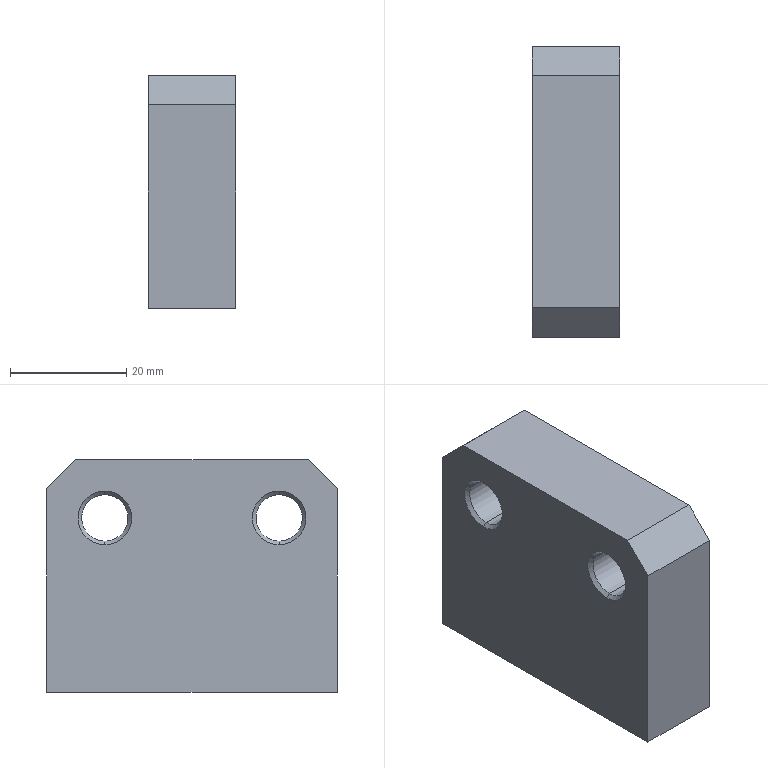Component | SolidWorks | DoubleFilmTransport-1_PositioningScrewPlate-1 | 1 solid | 28 faces | box 15 x 50 x 40 mm | volume 27415 mm3 | cone 12 | cylinder 8 | plane 8 | commonest cylinder face diameters 5 x4 8 x4
build123d program:
from build123d import *

# Parameters (mm, degrees)
SKETCH1_W                    = 40
SKETCH1_H                    = 50
BOSS_EXTRUDE1_DEPTH          = 15
F_6_8_6_8_DIAMETER_HOLE1_D   = 8
F_5_0_5_DIAMETER_HOLE1_D     = 5
F_5_0_5_DIAMETER_HOLE1_DEPTH = 17
F_5_0_5_DIAMETER_HOLE1_TIP   = 1.502
CHAMFER1_SIZE                = 0.625
CHAMFER2_SIZE                = 0.525
CHAMFER3_SIZE                = 5


with BuildPart() as part:
    # Sketch1 → Boss-Extrude1 (new body)
    with BuildSketch(Plane.XY.offset(7.5)):
        with Locations((20, 0)):
            Rectangle(SKETCH1_W, SKETCH1_H)
    extrude(amount=-BOSS_EXTRUDE1_DEPTH)

    # 6.8 _6.8_ Diameter Hole1 (through all)
    with Locations(Plane.XY.offset(7.5)):
        with Locations((30, -15), (30, 15)):
            Hole(F_6_8_6_8_DIAMETER_HOLE1_D / 2)

    # 5.0 _5_ Diameter Hole1
    with Locations(Plane.ZY):
        with Locations((0, -15), (0, 15)):
            Hole(F_5_0_5_DIAMETER_HOLE1_D / 2, depth=F_5_0_5_DIAMETER_HOLE1_DEPTH)
            with Locations((0, 0, -(F_5_0_5_DIAMETER_HOLE1_DEPTH + F_5_0_5_DIAMETER_HOLE1_TIP / 2))):  # 118° drill point
                Cone(0, F_5_0_5_DIAMETER_HOLE1_D / 2, F_5_0_5_DIAMETER_HOLE1_TIP, mode=Mode.SUBTRACT)

    # Chamfer1
    chamfer1_edges = [part.edges().sort_by_distance(p)[0] for p in [
        (34, 15, 7.5),
        (34, -15, 7.5),
    ]]
    chamfer(chamfer1_edges, length=CHAMFER1_SIZE)

    # Chamfer2
    chamfer2_edges = [part.edges().sort_by_distance(p)[0] for p in [
        (0, 15, 2.5),
        (0, -15, 2.5),
    ]]
    chamfer(chamfer2_edges, length=CHAMFER2_SIZE)

    # Chamfer3
    chamfer3_edges = [part.edges().sort_by_distance(p)[0] for p in [
        (40, 25, 0),
        (40, -25, 0),
    ]]
    chamfer(chamfer3_edges, length=CHAMFER3_SIZE)


solid = part.part

# Placed as in the assembly
solid = solid.moved(Location((-298.746, 150.373, -16.5), (0, -90, 0)))
STEP:
#1=CARTESIAN_POINT('',(-11.663,5.33,-0.6289));
#2=VERTEX_POINT('',#1);
#3=CARTESIAN_POINT('',(-11.86,5.33,-0.6289));
#4=VERTEX_POINT('',#3);
#5=CARTESIAN_POINT('',(-11.762,5.33,-0.6289));
#6=DIRECTION('',(0.,0.,-1.));
#7=DIRECTION('',(-1.,0.,0.));
#8=AXIS2_PLACEMENT_3D('',#5,#6,#7);
#9=CIRCLE('',#8,0.09843);
#10=EDGE_CURVE('',#2,#4,#9,.T.);
#11=ORIENTED_EDGE('',*,*,#10,.F.);
#12=CARTESIAN_POINT('',(-11.643,5.33,-0.6496));
#13=VERTEX_POINT('',#12);
#14=CARTESIAN_POINT('',(-11.663,5.33,-0.6289));
#15=DIRECTION('',(0.7071,0.,-0.7071));
#16=VECTOR('',#15,39.37);
#17=LINE('',#14,#16);
#18=EDGE_CURVE('',#2,#13,#17,.T.);
#19=ORIENTED_EDGE('',*,*,#18,.T.);
#20=CARTESIAN_POINT('',(-11.881,5.33,-0.6496));
#21=VERTEX_POINT('',#20);
#22=CARTESIAN_POINT('',(-11.762,5.33,-0.6496));
#23=DIRECTION('',(0.,-0.,1.));
#24=DIRECTION('',(0.,-1.,0.));
#25=AXIS2_PLACEMENT_3D('',#22,#23,#24);
#26=CIRCLE('',#25,0.1191);
#27=EDGE_CURVE('',#21,#13,#26,.T.);
#28=ORIENTED_EDGE('',*,*,#27,.F.);
#29=CARTESIAN_POINT('',(-11.86,5.33,-0.6289));
#30=DIRECTION('',(-0.7071,0.,-0.7071));
#31=VECTOR('',#30,39.37);
#32=LINE('',#29,#31);
#33=EDGE_CURVE('',#4,#21,#32,.T.);
#34=ORIENTED_EDGE('',*,*,#33,.F.);
#35=EDGE_LOOP('',(#11,#19,#28,#34));
#36=FACE_OUTER_BOUND('',#35,.T.);
#37=CARTESIAN_POINT('',(-11.762,5.33,-0.6289));
#38=DIRECTION('',(0.,0.,-1.));
#39=DIRECTION('',(-1.,0.,0.));
#40=AXIS2_PLACEMENT_3D('',#37,#38,#39);
#41=CONICAL_SURFACE('',#40,0.09843,0.7854);
#42=ADVANCED_FACE('',(#36),#41,.F.);
#43=CARTESIAN_POINT('',(-11.663,6.511,-0.6289));
#44=VERTEX_POINT('',#43);
#45=CARTESIAN_POINT('',(-11.86,6.511,-0.6289));
#46=VERTEX_POINT('',#45);
#47=CARTESIAN_POINT('',(-11.762,6.511,-0.6289));
#48=DIRECTION('',(0.,0.,-1.));
#49=DIRECTION('',(-1.,0.,0.));
#50=AXIS2_PLACEMENT_3D('',#47,#48,#49);
#51=CIRCLE('',#50,0.09843);
#52=EDGE_CURVE('',#44,#46,#51,.T.);
#53=ORIENTED_EDGE('',*,*,#52,.F.);
#54=CARTESIAN_POINT('',(-11.643,6.511,-0.6496));
#55=VERTEX_POINT('',#54);
#56=CARTESIAN_POINT('',(-11.663,6.511,-0.6289));
#57=DIRECTION('',(0.7071,0.,-0.7071));
#58=VECTOR('',#57,39.37);
#59=LINE('',#56,#58);
#60=EDGE_CURVE('',#44,#55,#59,.T.);
#61=ORIENTED_EDGE('',*,*,#60,.T.);
#62=CARTESIAN_POINT('',(-11.881,6.511,-0.6496));
#63=VERTEX_POINT('',#62);
#64=CARTESIAN_POINT('',(-11.762,6.511,-0.6496));
#65=DIRECTION('',(0.,-0.,1.));
#66=DIRECTION('',(0.,-1.,0.));
#67=AXIS2_PLACEMENT_3D('',#64,#65,#66);
#68=CIRCLE('',#67,0.1191);
#69=EDGE_CURVE('',#63,#55,#68,.T.);
#70=ORIENTED_EDGE('',*,*,#69,.F.);
#71=CARTESIAN_POINT('',(-11.86,6.511,-0.6289));
#72=DIRECTION('',(-0.7071,0.,-0.7071));
#73=VECTOR('',#72,39.37);
#74=LINE('',#71,#73);
#75=EDGE_CURVE('',#46,#63,#74,.T.);
#76=ORIENTED_EDGE('',*,*,#75,.F.);
#77=EDGE_LOOP('',(#53,#61,#70,#76));
#78=FACE_OUTER_BOUND('',#77,.T.);
#79=CARTESIAN_POINT('',(-11.762,6.511,-0.6289));
#80=DIRECTION('',(0.,0.,-1.));
#81=DIRECTION('',(-1.,0.,0.));
#82=AXIS2_PLACEMENT_3D('',#79,#80,#81);
#83=CONICAL_SURFACE('',#82,0.09843,0.7854);
#84=ADVANCED_FACE('',(#78),#83,.F.);
#85=CARTESIAN_POINT('',(-12.032,5.33,0.374));
#86=VERTEX_POINT('',#85);
#87=CARTESIAN_POINT('',(-12.032,5.33,0.689));
#88=VERTEX_POINT('',#87);
#89=CARTESIAN_POINT('',(-12.032,5.33,0.5315));
#90=DIRECTION('',(-1.,0.,0.));
#91=DIRECTION('',(0.,0.,1.));
#92=AXIS2_PLACEMENT_3D('',#89,#90,#91);
#93=CIRCLE('',#92,0.1575);
#94=EDGE_CURVE('',#86,#88,#93,.T.);
#95=ORIENTED_EDGE('',*,*,#94,.F.);
#96=CARTESIAN_POINT('',(-12.057,5.33,0.3494));
#97=VERTEX_POINT('',#96);
#98=CARTESIAN_POINT('',(-12.032,5.33,0.374));
#99=DIRECTION('',(-0.7071,0.,-0.7071));
#100=VECTOR('',#99,39.37);
#101=LINE('',#98,#100);
#102=EDGE_CURVE('',#86,#97,#101,.T.);
#103=ORIENTED_EDGE('',*,*,#102,.T.);
#104=CARTESIAN_POINT('',(-12.057,5.33,0.7136));
#105=VERTEX_POINT('',#104);
#106=CARTESIAN_POINT('',(-12.057,5.33,0.5315));
#107=DIRECTION('',(1.,0.,0.));
#108=DIRECTION('',(0.,0.,1.));
#109=AXIS2_PLACEMENT_3D('',#106,#107,#108);
#110=CIRCLE('',#109,0.1821);
#111=EDGE_CURVE('',#105,#97,#110,.T.);
#112=ORIENTED_EDGE('',*,*,#111,.F.);
#113=CARTESIAN_POINT('',(-12.032,5.33,0.689));
#114=DIRECTION('',(-0.7071,0.,0.7071));
#115=VECTOR('',#114,39.37);
#116=LINE('',#113,#115);
#117=EDGE_CURVE('',#88,#105,#116,.T.);
#118=ORIENTED_EDGE('',*,*,#117,.F.);
#119=EDGE_LOOP('',(#95,#103,#112,#118));
#120=FACE_OUTER_BOUND('',#119,.T.);
#121=CARTESIAN_POINT('',(-12.032,5.33,0.5315));
#122=DIRECTION('',(-1.,0.,0.));
#123=DIRECTION('',(0.,0.,1.));
#124=AXIS2_PLACEMENT_3D('',#121,#122,#123);
#125=CONICAL_SURFACE('',#124,0.1575,0.7854);
#126=ADVANCED_FACE('',(#120),#125,.F.);
#127=CARTESIAN_POINT('',(-12.032,6.511,0.374));
#128=VERTEX_POINT('',#127);
#129=CARTESIAN_POINT('',(-12.032,6.511,0.689));
#130=VERTEX_POINT('',#129);
#131=CARTESIAN_POINT('',(-12.032,6.511,0.5315));
#132=DIRECTION('',(-1.,0.,0.));
#133=DIRECTION('',(0.,0.,1.));
#134=AXIS2_PLACEMENT_3D('',#131,#132,#133);
#135=CIRCLE('',#134,0.1575);
#136=EDGE_CURVE('',#128,#130,#135,.T.);
#137=ORIENTED_EDGE('',*,*,#136,.F.);
#138=CARTESIAN_POINT('',(-12.057,6.511,0.3494));
#139=VERTEX_POINT('',#138);
#140=CARTESIAN_POINT('',(-12.032,6.511,0.374));
#141=DIRECTION('',(-0.7071,0.,-0.7071));
#142=VECTOR('',#141,39.37);
#143=LINE('',#140,#142);
#144=EDGE_CURVE('',#128,#139,#143,.T.);
#145=ORIENTED_EDGE('',*,*,#144,.T.);
#146=CARTESIAN_POINT('',(-12.057,6.511,0.7136));
#147=VERTEX_POINT('',#146);
#148=CARTESIAN_POINT('',(-12.057,6.511,0.5315));
#149=DIRECTION('',(1.,0.,0.));
#150=DIRECTION('',(0.,0.,1.));
#151=AXIS2_PLACEMENT_3D('',#148,#149,#150);
#152=CIRCLE('',#151,0.1821);
#153=EDGE_CURVE('',#147,#139,#152,.T.);
#154=ORIENTED_EDGE('',*,*,#153,.F.);
#155=CARTESIAN_POINT('',(-12.032,6.511,0.689));
#156=DIRECTION('',(-0.7071,0.,0.7071));
#157=VECTOR('',#156,39.37);
#158=LINE('',#155,#157);
#159=EDGE_CURVE('',#130,#147,#158,.T.);
#160=ORIENTED_EDGE('',*,*,#159,.F.);
#161=EDGE_LOOP('',(#137,#145,#154,#160));
#162=FACE_OUTER_BOUND('',#161,.T.);
#163=CARTESIAN_POINT('',(-12.032,6.511,0.5315));
#164=DIRECTION('',(-1.,0.,0.));
#165=DIRECTION('',(0.,0.,1.));
#166=AXIS2_PLACEMENT_3D('',#163,#164,#165);
#167=CONICAL_SURFACE('',#166,0.1575,0.7854);
#168=ADVANCED_FACE('',(#162),#167,.F.);
#169=CARTESIAN_POINT('',(-11.663,5.33,0.01969));
#170=VERTEX_POINT('',#169);
#171=CARTESIAN_POINT('',(-11.86,5.33,0.01969));
#172=VERTEX_POINT('',#171);
#173=CARTESIAN_POINT('',(-11.762,5.33,0.01969));
#174=DIRECTION('',(0.,0.,-1.));
#175=DIRECTION('',(-1.,0.,0.));
#176=AXIS2_PLACEMENT_3D('',#173,#174,#175);
#177=CIRCLE('',#176,0.09843);
#178=EDGE_CURVE('',#170,#172,#177,.T.);
#179=ORIENTED_EDGE('',*,*,#178,.F.);
#180=CARTESIAN_POINT('',(-11.663,5.33,-0.6496));
#181=DIRECTION('',(0.,0.,-1.));
#182=VECTOR('',#181,39.37);
#183=LINE('',#180,#182);
#184=EDGE_CURVE('',#170,#2,#183,.T.);
#185=ORIENTED_EDGE('',*,*,#184,.T.);
#186=ORIENTED_EDGE('',*,*,#10,.T.);
#187=CARTESIAN_POINT('',(-11.86,5.33,-0.6496));
#188=DIRECTION('',(0.,0.,-1.));
#189=VECTOR('',#188,39.37);
#190=LINE('',#187,#189);
#191=EDGE_CURVE('',#172,#4,#190,.T.);
#192=ORIENTED_EDGE('',*,*,#191,.F.);
#193=EDGE_LOOP('',(#179,#185,#186,#192));
#194=FACE_OUTER_BOUND('',#193,.T.);
#195=CARTESIAN_POINT('',(-11.762,5.33,-0.6496));
#196=DIRECTION('',(0.,0.,-1.));
#197=DIRECTION('',(-1.,0.,0.));
#198=AXIS2_PLACEMENT_3D('',#195,#196,#197);
#199=CYLINDRICAL_SURFACE('',#198,0.09843);
#200=ADVANCED_FACE('',(#194),#199,.F.);
#201=CARTESIAN_POINT('',(-11.762,5.33,0.07882));
#202=VERTEX_POINT('',#201);
#203=CARTESIAN_POINT('',(-11.86,5.33,0.01969));
#204=DIRECTION('',(-0.8572,0.,-0.515));
#205=VECTOR('',#204,39.37);
#206=LINE('',#203,#205);
#207=EDGE_CURVE('',#202,#172,#206,.T.);
#208=ORIENTED_EDGE('',*,*,#207,.F.);
#209=CARTESIAN_POINT('',(-11.663,5.33,0.01969));
#210=DIRECTION('',(0.8572,0.,-0.515));
#211=VECTOR('',#210,39.37);
#212=LINE('',#209,#211);
#213=EDGE_CURVE('',#202,#170,#212,.T.);
#214=ORIENTED_EDGE('',*,*,#213,.T.);
#215=ORIENTED_EDGE('',*,*,#178,.T.);
#216=EDGE_LOOP('',(#208,#214,#215));
#217=FACE_OUTER_BOUND('',#216,.T.);
#218=CARTESIAN_POINT('',(-11.762,5.33,0.01969));
#219=DIRECTION('',(0.,0.,-1.));
#220=DIRECTION('',(-1.,0.,0.));
#221=AXIS2_PLACEMENT_3D('',#218,#219,#220);
#222=CONICAL_SURFACE('',#221,0.09843,1.03);
#223=ADVANCED_FACE('',(#217),#222,.F.);
#224=CARTESIAN_POINT('',(-11.663,6.511,0.01969));
#225=VERTEX_POINT('',#224);
#226=CARTESIAN_POINT('',(-11.86,6.511,0.01969));
#227=VERTEX_POINT('',#226);
#228=CARTESIAN_POINT('',(-11.762,6.511,0.01969));
#229=DIRECTION('',(0.,0.,-1.));
#230=DIRECTION('',(-1.,0.,0.));
#231=AXIS2_PLACEMENT_3D('',#228,#229,#230);
#232=CIRCLE('',#231,0.09843);
#233=EDGE_CURVE('',#225,#227,#232,.T.);
#234=ORIENTED_EDGE('',*,*,#233,.F.);
#235=CARTESIAN_POINT('',(-11.663,6.511,-0.6496));
#236=DIRECTION('',(0.,0.,-1.));
#237=VECTOR('',#236,39.37);
#238=LINE('',#235,#237);
#239=EDGE_CURVE('',#225,#44,#238,.T.);
#240=ORIENTED_EDGE('',*,*,#239,.T.);
#241=ORIENTED_EDGE('',*,*,#52,.T.);
#242=CARTESIAN_POINT('',(-11.86,6.511,-0.6496));
#243=DIRECTION('',(0.,0.,-1.));
#244=VECTOR('',#243,39.37);
#245=LINE('',#242,#244);
#246=EDGE_CURVE('',#227,#46,#245,.T.);
#247=ORIENTED_EDGE('',*,*,#246,.F.);
#248=EDGE_LOOP('',(#234,#240,#241,#247));
#249=FACE_OUTER_BOUND('',#248,.T.);
#250=CARTESIAN_POINT('',(-11.762,6.511,-0.6496));
#251=DIRECTION('',(0.,0.,-1.));
#252=DIRECTION('',(-1.,0.,0.));
#253=AXIS2_PLACEMENT_3D('',#250,#251,#252);
#254=CYLINDRICAL_SURFACE('',#253,0.09843);
#255=ADVANCED_FACE('',(#249),#254,.F.);
#256=CARTESIAN_POINT('',(-11.762,6.511,0.07882));
#257=VERTEX_POINT('',#256);
#258=CARTESIAN_POINT('',(-11.86,6.511,0.01969));
#259=DIRECTION('',(-0.8572,0.,-0.515));
#260=VECTOR('',#259,39.37);
#261=LINE('',#258,#260);
#262=EDGE_CURVE('',#257,#227,#261,.T.);
#263=ORIENTED_EDGE('',*,*,#262,.F.);
#264=CARTESIAN_POINT('',(-11.663,6.511,0.01969));
#265=DIRECTION('',(0.8572,0.,-0.515));
#266=VECTOR('',#265,39.37);
#267=LINE('',#264,#266);
#268=EDGE_CURVE('',#257,#225,#267,.T.);
#269=ORIENTED_EDGE('',*,*,#268,.T.);
#270=ORIENTED_EDGE('',*,*,#233,.T.);
#271=EDGE_LOOP('',(#263,#269,#270));
#272=FACE_OUTER_BOUND('',#271,.T.);
#273=CARTESIAN_POINT('',(-11.762,6.511,0.01969));
#274=DIRECTION('',(0.,0.,-1.));
#275=DIRECTION('',(-1.,0.,0.));
#276=AXIS2_PLACEMENT_3D('',#273,#274,#275);
#277=CONICAL_SURFACE('',#276,0.09843,1.03);
#278=ADVANCED_FACE('',(#272),#277,.F.);
#279=CARTESIAN_POINT('',(-11.466,5.33,0.374));
#280=VERTEX_POINT('',#279);
#281=CARTESIAN_POINT('',(-11.466,5.33,0.689));
#282=VERTEX_POINT('',#281);
#283=CARTESIAN_POINT('',(-11.466,5.33,0.5315));
#284=DIRECTION('',(-1.,0.,0.));
#285=DIRECTION('',(0.,0.,1.));
#286=AXIS2_PLACEMENT_3D('',#283,#284,#285);
#287=CIRCLE('',#286,0.1575);
#288=EDGE_CURVE('',#280,#282,#287,.T.);
#289=ORIENTED_EDGE('',*,*,#288,.F.);
#290=CARTESIAN_POINT('',(-12.057,5.33,0.374));
#291=DIRECTION('',(-1.,0.,0.));
#292=VECTOR('',#291,39.37);
#293=LINE('',#290,#292);
#294=EDGE_CURVE('',#280,#86,#293,.T.);
#295=ORIENTED_EDGE('',*,*,#294,.T.);
#296=ORIENTED_EDGE('',*,*,#94,.T.);
#297=CARTESIAN_POINT('',(-12.057,5.33,0.689));
#298=DIRECTION('',(-1.,0.,0.));
#299=VECTOR('',#298,39.37);
#300=LINE('',#297,#299);
#301=EDGE_CURVE('',#282,#88,#300,.T.);
#302=ORIENTED_EDGE('',*,*,#301,.F.);
#303=EDGE_LOOP('',(#289,#295,#296,#302));
#304=FACE_OUTER_BOUND('',#303,.T.);
#305=CARTESIAN_POINT('',(-12.057,5.33,0.5315));
#306=DIRECTION('',(-1.,0.,0.));
#307=DIRECTION('',(0.,0.,1.));
#308=AXIS2_PLACEMENT_3D('',#305,#306,#307);
#309=CYLINDRICAL_SURFACE('',#308,0.1575);
#310=ADVANCED_FACE('',(#304),#309,.F.);
#311=CARTESIAN_POINT('',(-11.466,6.511,0.374));
#312=VERTEX_POINT('',#311);
#313=CARTESIAN_POINT('',(-11.466,6.511,0.689));
#314=VERTEX_POINT('',#313);
#315=CARTESIAN_POINT('',(-11.466,6.511,0.5315));
#316=DIRECTION('',(-1.,0.,0.));
#317=DIRECTION('',(0.,0.,1.));
#318=AXIS2_PLACEMENT_3D('',#315,#316,#317);
#319=CIRCLE('',#318,0.1575);
#320=EDGE_CURVE('',#312,#314,#319,.T.);
#321=ORIENTED_EDGE('',*,*,#320,.F.);
#322=CARTESIAN_POINT('',(-12.057,6.511,0.374));
#323=DIRECTION('',(-1.,0.,0.));
#324=VECTOR('',#323,39.37);
#325=LINE('',#322,#324);
#326=EDGE_CURVE('',#312,#128,#325,.T.);
#327=ORIENTED_EDGE('',*,*,#326,.T.);
#328=ORIENTED_EDGE('',*,*,#136,.T.);
#329=CARTESIAN_POINT('',(-12.057,6.511,0.689));
#330=DIRECTION('',(-1.,0.,0.));
#331=VECTOR('',#330,39.37);
#332=LINE('',#329,#331);
#333=EDGE_CURVE('',#314,#130,#332,.T.);
#334=ORIENTED_EDGE('',*,*,#333,.F.);
#335=EDGE_LOOP('',(#321,#327,#328,#334));
#336=FACE_OUTER_BOUND('',#335,.T.);
#337=CARTESIAN_POINT('',(-12.057,6.511,0.5315));
#338=DIRECTION('',(-1.,0.,0.));
#339=DIRECTION('',(0.,0.,1.));
#340=AXIS2_PLACEMENT_3D('',#337,#338,#339);
#341=CYLINDRICAL_SURFACE('',#340,0.1575);
#342=ADVANCED_FACE('',(#336),#341,.F.);
#343=ORIENTED_EDGE('',*,*,#69,.T.);
#344=CARTESIAN_POINT('',(-11.762,6.511,-0.6496));
#345=DIRECTION('',(0.,-0.,1.));
#346=DIRECTION('',(0.,-1.,0.));
#347=AXIS2_PLACEMENT_3D('',#344,#345,#346);
#348=CIRCLE('',#347,0.1191);
#349=EDGE_CURVE('',#55,#63,#348,.T.);
#350=ORIENTED_EDGE('',*,*,#349,.T.);
#351=EDGE_LOOP('',(#343,#350));
#352=FACE_BOUND('',#351,.T.);
#353=ORIENTED_EDGE('',*,*,#27,.T.);
#354=CARTESIAN_POINT('',(-11.762,5.33,-0.6496));
#355=DIRECTION('',(0.,-0.,1.));
#356=DIRECTION('',(0.,-1.,0.));
#357=AXIS2_PLACEMENT_3D('',#354,#355,#356);
#358=CIRCLE('',#357,0.1191);
#359=EDGE_CURVE('',#13,#21,#358,.T.);
#360=ORIENTED_EDGE('',*,*,#359,.T.);
#361=EDGE_LOOP('',(#353,#360));
#362=FACE_BOUND('',#361,.T.);
#363=CARTESIAN_POINT('',(-12.057,6.904,-0.6496));
#364=VERTEX_POINT('',#363);
#365=CARTESIAN_POINT('',(-12.057,4.936,-0.6496));
#366=VERTEX_POINT('',#365);
#367=CARTESIAN_POINT('',(-12.057,6.904,-0.6496));
#368=DIRECTION('',(0.,-1.,-0.));
#369=VECTOR('',#368,39.37);
#370=LINE('',#367,#369);
#371=EDGE_CURVE('',#364,#366,#370,.T.);
#372=ORIENTED_EDGE('',*,*,#371,.F.);
#373=CARTESIAN_POINT('',(-11.466,6.904,-0.6496));
#374=VERTEX_POINT('',#373);
#375=CARTESIAN_POINT('',(-11.466,6.904,-0.6496));
#376=DIRECTION('',(-1.,0.,0.));
#377=VECTOR('',#376,39.37);
#378=LINE('',#375,#377);
#379=EDGE_CURVE('',#374,#364,#378,.T.);
#380=ORIENTED_EDGE('',*,*,#379,.F.);
#381=CARTESIAN_POINT('',(-11.466,4.936,-0.6496));
#382=VERTEX_POINT('',#381);
#383=CARTESIAN_POINT('',(-11.466,6.904,-0.6496));
#384=DIRECTION('',(0.,-1.,-0.));
#385=VECTOR('',#384,39.37);
#386=LINE('',#383,#385);
#387=EDGE_CURVE('',#374,#382,#386,.T.);
#388=ORIENTED_EDGE('',*,*,#387,.T.);
#389=CARTESIAN_POINT('',(-11.466,4.936,-0.6496));
#390=DIRECTION('',(-1.,0.,0.));
#391=VECTOR('',#390,39.37);
#392=LINE('',#389,#391);
#393=EDGE_CURVE('',#382,#366,#392,.T.);
#394=ORIENTED_EDGE('',*,*,#393,.T.);
#395=EDGE_LOOP('',(#372,#380,#388,#394));
#396=FACE_OUTER_BOUND('',#395,.T.);
#397=CARTESIAN_POINT('',(-11.466,6.904,-0.6496));
#398=DIRECTION('',(0.,0.,-1.));
#399=DIRECTION('',(0.,-1.,-0.));
#400=AXIS2_PLACEMENT_3D('',#397,#398,#399);
#401=PLANE('',#400);
#402=ADVANCED_FACE('',(#352,#362,#396),#401,.T.);
#403=CARTESIAN_POINT('',(-12.057,6.904,0.7283));
#404=VERTEX_POINT('',#403);
#405=CARTESIAN_POINT('',(-12.057,6.904,0.9252));
#406=DIRECTION('',(0.,0.,-1.));
#407=VECTOR('',#406,39.37);
#408=LINE('',#405,#407);
#409=EDGE_CURVE('',#404,#364,#408,.T.);
#410=ORIENTED_EDGE('',*,*,#409,.F.);
#411=CARTESIAN_POINT('',(-11.466,6.904,0.7283));
#412=VERTEX_POINT('',#411);
#413=CARTESIAN_POINT('',(-11.466,6.904,0.7283));
#414=DIRECTION('',(1.,0.,0.));
#415=VECTOR('',#414,39.37);
#416=LINE('',#413,#415);
#417=EDGE_CURVE('',#404,#412,#416,.T.);
#418=ORIENTED_EDGE('',*,*,#417,.T.);
#419=CARTESIAN_POINT('',(-11.466,6.904,0.9252));
#420=DIRECTION('',(0.,0.,-1.));
#421=VECTOR('',#420,39.37);
#422=LINE('',#419,#421);
#423=EDGE_CURVE('',#412,#374,#422,.T.);
#424=ORIENTED_EDGE('',*,*,#423,.T.);
#425=ORIENTED_EDGE('',*,*,#379,.T.);
#426=EDGE_LOOP('',(#410,#418,#424,#425));
#427=FACE_OUTER_BOUND('',#426,.T.);
#428=CARTESIAN_POINT('',(-11.466,6.904,0.9252));
#429=DIRECTION('',(0.,1.,0.));
#430=DIRECTION('',(-1.,0.,0.));
#431=AXIS2_PLACEMENT_3D('',#428,#429,#430);
#432=PLANE('',#431);
#433=ADVANCED_FACE('',(#427),#432,.T.);
#434=CARTESIAN_POINT('',(-11.466,5.133,0.9252));
#435=VERTEX_POINT('',#434);
#436=CARTESIAN_POINT('',(-11.466,6.708,0.9252));
#437=VERTEX_POINT('',#436);
#438=CARTESIAN_POINT('',(-11.466,4.936,0.9252));
#439=DIRECTION('',(0.,1.,0.));
#440=VECTOR('',#439,39.37);
#441=LINE('',#438,#440);
#442=EDGE_CURVE('',#435,#437,#441,.T.);
#443=ORIENTED_EDGE('',*,*,#442,.T.);
#444=CARTESIAN_POINT('',(-12.057,6.708,0.9252));
#445=VERTEX_POINT('',#444);
#446=CARTESIAN_POINT('',(-11.466,6.708,0.9252));
#447=DIRECTION('',(-1.,0.,0.));
#448=VECTOR('',#447,39.37);
#449=LINE('',#446,#448);
#450=EDGE_CURVE('',#437,#445,#449,.T.);
#451=ORIENTED_EDGE('',*,*,#450,.T.);
#452=CARTESIAN_POINT('',(-12.057,5.133,0.9252));
#453=VERTEX_POINT('',#452);
#454=CARTESIAN_POINT('',(-12.057,4.936,0.9252));
#455=DIRECTION('',(0.,1.,0.));
#456=VECTOR('',#455,39.37);
#457=LINE('',#454,#456);
#458=EDGE_CURVE('',#453,#445,#457,.T.);
#459=ORIENTED_EDGE('',*,*,#458,.F.);
#460=CARTESIAN_POINT('',(-11.466,5.133,0.9252));
#461=DIRECTION('',(1.,0.,0.));
#462=VECTOR('',#461,39.37);
#463=LINE('',#460,#462);
#464=EDGE_CURVE('',#453,#435,#463,.T.);
#465=ORIENTED_EDGE('',*,*,#464,.T.);
#466=EDGE_LOOP('',(#443,#451,#459,#465));
#467=FACE_OUTER_BOUND('',#466,.T.);
#468=CARTESIAN_POINT('',(-11.466,4.936,0.9252));
#469=DIRECTION('',(0.,-0.,1.));
#470=DIRECTION('',(0.,1.,0.));
#471=AXIS2_PLACEMENT_3D('',#468,#469,#470);
#472=PLANE('',#471);
#473=ADVANCED_FACE('',(#467),#472,.T.);
#474=CARTESIAN_POINT('',(-11.466,4.936,0.7283));
#475=VERTEX_POINT('',#474);
#476=CARTESIAN_POINT('',(-11.466,4.936,-0.6496));
#477=DIRECTION('',(0.,0.,1.));
#478=VECTOR('',#477,39.37);
#479=LINE('',#476,#478);
#480=EDGE_CURVE('',#382,#475,#479,.T.);
#481=ORIENTED_EDGE('',*,*,#480,.T.);
#482=CARTESIAN_POINT('',(-12.057,4.936,0.7283));
#483=VERTEX_POINT('',#482);
#484=CARTESIAN_POINT('',(-11.466,4.936,0.7283));
#485=DIRECTION('',(-1.,0.,0.));
#486=VECTOR('',#485,39.37);
#487=LINE('',#484,#486);
#488=EDGE_CURVE('',#475,#483,#487,.T.);
#489=ORIENTED_EDGE('',*,*,#488,.T.);
#490=CARTESIAN_POINT('',(-12.057,4.936,-0.6496));
#491=DIRECTION('',(0.,0.,1.));
#492=VECTOR('',#491,39.37);
#493=LINE('',#490,#492);
#494=EDGE_CURVE('',#366,#483,#493,.T.);
#495=ORIENTED_EDGE('',*,*,#494,.F.);
#496=ORIENTED_EDGE('',*,*,#393,.F.);
#497=EDGE_LOOP('',(#481,#489,#495,#496));
#498=FACE_OUTER_BOUND('',#497,.T.);
#499=CARTESIAN_POINT('',(-11.466,4.936,-0.6496));
#500=DIRECTION('',(0.,-1.,0.));
#501=DIRECTION('',(1.,0.,0.));
#502=AXIS2_PLACEMENT_3D('',#499,#500,#501);
#503=PLANE('',#502);
#504=ADVANCED_FACE('',(#498),#503,.T.);
#505=CARTESIAN_POINT('',(-11.466,5.33,0.5315));
#506=DIRECTION('',(-1.,0.,0.));
#507=DIRECTION('',(0.,0.,1.));
#508=AXIS2_PLACEMENT_3D('',#505,#506,#507);
#509=CIRCLE('',#508,0.1575);
#510=EDGE_CURVE('',#282,#280,#509,.T.);
#511=ORIENTED_EDGE('',*,*,#510,.T.);
#512=ORIENTED_EDGE('',*,*,#288,.T.);
#513=EDGE_LOOP('',(#511,#512));
#514=FACE_BOUND('',#513,.T.);
#515=CARTESIAN_POINT('',(-11.466,6.511,0.5315));
#516=DIRECTION('',(-1.,0.,0.));
#517=DIRECTION('',(0.,0.,1.));
#518=AXIS2_PLACEMENT_3D('',#515,#516,#517);
#519=CIRCLE('',#518,0.1575);
#520=EDGE_CURVE('',#314,#312,#519,.T.);
#521=ORIENTED_EDGE('',*,*,#520,.T.);
#522=ORIENTED_EDGE('',*,*,#320,.T.);
#523=EDGE_LOOP('',(#521,#522));
#524=FACE_BOUND('',#523,.T.);
#525=ORIENTED_EDGE('',*,*,#423,.F.);
#526=CARTESIAN_POINT('',(-11.466,6.708,0.9252));
#527=DIRECTION('',(0.,-0.7071,0.7071));
#528=VECTOR('',#527,39.37);
#529=LINE('',#526,#528);
#530=EDGE_CURVE('',#412,#437,#529,.T.);
#531=ORIENTED_EDGE('',*,*,#530,.T.);
#532=ORIENTED_EDGE('',*,*,#442,.F.);
#533=CARTESIAN_POINT('',(-11.466,4.936,0.7283));
#534=DIRECTION('',(0.,-0.7071,-0.7071));
#535=VECTOR('',#534,39.37);
#536=LINE('',#533,#535);
#537=EDGE_CURVE('',#435,#475,#536,.T.);
#538=ORIENTED_EDGE('',*,*,#537,.T.);
#539=ORIENTED_EDGE('',*,*,#480,.F.);
#540=ORIENTED_EDGE('',*,*,#387,.F.);
#541=EDGE_LOOP('',(#525,#531,#532,#538,#539,#540));
#542=FACE_OUTER_BOUND('',#541,.T.);
#543=CARTESIAN_POINT('',(-11.466,5.92,-0.6496));
#544=DIRECTION('',(-1.,0.,0.));
#545=DIRECTION('',(0.,0.,1.));
#546=AXIS2_PLACEMENT_3D('',#543,#544,#545);
#547=PLANE('',#546);
#548=ADVANCED_FACE('',(#514,#524,#542),#547,.F.);
#549=ORIENTED_EDGE('',*,*,#153,.T.);
#550=CARTESIAN_POINT('',(-12.057,6.511,0.5315));
#551=DIRECTION('',(1.,0.,0.));
#552=DIRECTION('',(0.,0.,1.));
#553=AXIS2_PLACEMENT_3D('',#550,#551,#552);
#554=CIRCLE('',#553,0.1821);
#555=EDGE_CURVE('',#139,#147,#554,.T.);
#556=ORIENTED_EDGE('',*,*,#555,.T.);
#557=EDGE_LOOP('',(#549,#556));
#558=FACE_BOUND('',#557,.T.);
#559=ORIENTED_EDGE('',*,*,#111,.T.);
#560=CARTESIAN_POINT('',(-12.057,5.33,0.5315));
#561=DIRECTION('',(1.,0.,0.));
#562=DIRECTION('',(0.,0.,1.));
#563=AXIS2_PLACEMENT_3D('',#560,#561,#562);
#564=CIRCLE('',#563,0.1821);
#565=EDGE_CURVE('',#97,#105,#564,.T.);
#566=ORIENTED_EDGE('',*,*,#565,.T.);
#567=EDGE_LOOP('',(#559,#566));
#568=FACE_BOUND('',#567,.T.);
#569=ORIENTED_EDGE('',*,*,#458,.T.);
#570=CARTESIAN_POINT('',(-12.057,7.101,0.5315));
#571=DIRECTION('',(0.,0.7071,-0.7071));
#572=VECTOR('',#571,39.37);
#573=LINE('',#570,#572);
#574=EDGE_CURVE('',#445,#404,#573,.T.);
#575=ORIENTED_EDGE('',*,*,#574,.T.);
#576=ORIENTED_EDGE('',*,*,#409,.T.);
#577=ORIENTED_EDGE('',*,*,#371,.T.);
#578=ORIENTED_EDGE('',*,*,#494,.T.);
#579=CARTESIAN_POINT('',(-12.057,4.739,0.5315));
#580=DIRECTION('',(0.,0.7071,0.7071));
#581=VECTOR('',#580,39.37);
#582=LINE('',#579,#581);
#583=EDGE_CURVE('',#483,#453,#582,.T.);
#584=ORIENTED_EDGE('',*,*,#583,.T.);
#585=EDGE_LOOP('',(#569,#575,#576,#577,#578,#584));
#586=FACE_OUTER_BOUND('',#585,.T.);
#587=CARTESIAN_POINT('',(-12.057,5.92,-0.6496));
#588=DIRECTION('',(-1.,0.,0.));
#589=DIRECTION('',(0.,0.,1.));
#590=AXIS2_PLACEMENT_3D('',#587,#588,#589);
#591=PLANE('',#590);
#592=ADVANCED_FACE('',(#558,#568,#586),#591,.T.);
#593=ORIENTED_EDGE('',*,*,#326,.F.);
#594=ORIENTED_EDGE('',*,*,#520,.F.);
#595=ORIENTED_EDGE('',*,*,#333,.T.);
#596=CARTESIAN_POINT('',(-12.032,6.511,0.5315));
#597=DIRECTION('',(-1.,0.,0.));
#598=DIRECTION('',(0.,0.,1.));
#599=AXIS2_PLACEMENT_3D('',#596,#597,#598);
#600=CIRCLE('',#599,0.1575);
#601=EDGE_CURVE('',#130,#128,#600,.T.);
#602=ORIENTED_EDGE('',*,*,#601,.T.);
#603=EDGE_LOOP('',(#593,#594,#595,#602));
#604=FACE_OUTER_BOUND('',#603,.T.);
#605=CARTESIAN_POINT('',(-12.057,6.511,0.5315));
#606=DIRECTION('',(-1.,0.,0.));
#607=DIRECTION('',(0.,0.,1.));
#608=AXIS2_PLACEMENT_3D('',#605,#606,#607);
#609=CYLINDRICAL_SURFACE('',#608,0.1575);
#610=ADVANCED_FACE('',(#604),#609,.F.);
#611=ORIENTED_EDGE('',*,*,#294,.F.);
#612=ORIENTED_EDGE('',*,*,#510,.F.);
#613=ORIENTED_EDGE('',*,*,#301,.T.);
#614=CARTESIAN_POINT('',(-12.032,5.33,0.5315));
#615=DIRECTION('',(-1.,0.,0.));
#616=DIRECTION('',(0.,0.,1.));
#617=AXIS2_PLACEMENT_3D('',#614,#615,#616);
#618=CIRCLE('',#617,0.1575);
#619=EDGE_CURVE('',#88,#86,#618,.T.);
#620=ORIENTED_EDGE('',*,*,#619,.T.);
#621=EDGE_LOOP('',(#611,#612,#613,#620));
#622=FACE_OUTER_BOUND('',#621,.T.);
#623=CARTESIAN_POINT('',(-12.057,5.33,0.5315));
#624=DIRECTION('',(-1.,0.,0.));
#625=DIRECTION('',(0.,0.,1.));
#626=AXIS2_PLACEMENT_3D('',#623,#624,#625);
#627=CYLINDRICAL_SURFACE('',#626,0.1575);
#628=ADVANCED_FACE('',(#622),#627,.F.);
#629=ORIENTED_EDGE('',*,*,#268,.F.);
#630=ORIENTED_EDGE('',*,*,#262,.T.);
#631=CARTESIAN_POINT('',(-11.762,6.511,0.01969));
#632=DIRECTION('',(0.,0.,-1.));
#633=DIRECTION('',(-1.,0.,0.));
#634=AXIS2_PLACEMENT_3D('',#631,#632,#633);
#635=CIRCLE('',#634,0.09843);
#636=EDGE_CURVE('',#227,#225,#635,.T.);
#637=ORIENTED_EDGE('',*,*,#636,.T.);
#638=EDGE_LOOP('',(#629,#630,#637));
#639=FACE_OUTER_BOUND('',#638,.T.);
#640=CARTESIAN_POINT('',(-11.762,6.511,0.01969));
#641=DIRECTION('',(0.,0.,-1.));
#642=DIRECTION('',(-1.,0.,0.));
#643=AXIS2_PLACEMENT_3D('',#640,#641,#642);
#644=CONICAL_SURFACE('',#643,0.09843,1.03);
#645=ADVANCED_FACE('',(#639),#644,.F.);
#646=ORIENTED_EDGE('',*,*,#239,.F.);
#647=ORIENTED_EDGE('',*,*,#636,.F.);
#648=ORIENTED_EDGE('',*,*,#246,.T.);
#649=CARTESIAN_POINT('',(-11.762,6.511,-0.6289));
#650=DIRECTION('',(0.,0.,-1.));
#651=DIRECTION('',(-1.,0.,0.));
#652=AXIS2_PLACEMENT_3D('',#649,#650,#651);
#653=CIRCLE('',#652,0.09843);
#654=EDGE_CURVE('',#46,#44,#653,.T.);
#655=ORIENTED_EDGE('',*,*,#654,.T.);
#656=EDGE_LOOP('',(#646,#647,#648,#655));
#657=FACE_OUTER_BOUND('',#656,.T.);
#658=CARTESIAN_POINT('',(-11.762,6.511,-0.6496));
#659=DIRECTION('',(0.,0.,-1.));
#660=DIRECTION('',(-1.,0.,0.));
#661=AXIS2_PLACEMENT_3D('',#658,#659,#660);
#662=CYLINDRICAL_SURFACE('',#661,0.09843);
#663=ADVANCED_FACE('',(#657),#662,.F.);
#664=ORIENTED_EDGE('',*,*,#213,.F.);
#665=ORIENTED_EDGE('',*,*,#207,.T.);
#666=CARTESIAN_POINT('',(-11.762,5.33,0.01969));
#667=DIRECTION('',(0.,0.,-1.));
#668=DIRECTION('',(-1.,0.,0.));
#669=AXIS2_PLACEMENT_3D('',#666,#667,#668);
#670=CIRCLE('',#669,0.09843);
#671=EDGE_CURVE('',#172,#170,#670,.T.);
#672=ORIENTED_EDGE('',*,*,#671,.T.);
#673=EDGE_LOOP('',(#664,#665,#672));
#674=FACE_OUTER_BOUND('',#673,.T.);
#675=CARTESIAN_POINT('',(-11.762,5.33,0.01969));
#676=DIRECTION('',(0.,0.,-1.));
#677=DIRECTION('',(-1.,0.,0.));
#678=AXIS2_PLACEMENT_3D('',#675,#676,#677);
#679=CONICAL_SURFACE('',#678,0.09843,1.03);
#680=ADVANCED_FACE('',(#674),#679,.F.);
#681=ORIENTED_EDGE('',*,*,#184,.F.);
#682=ORIENTED_EDGE('',*,*,#671,.F.);
#683=ORIENTED_EDGE('',*,*,#191,.T.);
#684=CARTESIAN_POINT('',(-11.762,5.33,-0.6289));
#685=DIRECTION('',(0.,0.,-1.));
#686=DIRECTION('',(-1.,0.,0.));
#687=AXIS2_PLACEMENT_3D('',#684,#685,#686);
#688=CIRCLE('',#687,0.09843);
#689=EDGE_CURVE('',#4,#2,#688,.T.);
#690=ORIENTED_EDGE('',*,*,#689,.T.);
#691=EDGE_LOOP('',(#681,#682,#683,#690));
#692=FACE_OUTER_BOUND('',#691,.T.);
#693=CARTESIAN_POINT('',(-11.762,5.33,-0.6496));
#694=DIRECTION('',(0.,0.,-1.));
#695=DIRECTION('',(-1.,0.,0.));
#696=AXIS2_PLACEMENT_3D('',#693,#694,#695);
#697=CYLINDRICAL_SURFACE('',#696,0.09843);
#698=ADVANCED_FACE('',(#692),#697,.F.);
#699=ORIENTED_EDGE('',*,*,#144,.F.);
#700=ORIENTED_EDGE('',*,*,#601,.F.);
#701=ORIENTED_EDGE('',*,*,#159,.T.);
#702=ORIENTED_EDGE('',*,*,#555,.F.);
#703=EDGE_LOOP('',(#699,#700,#701,#702));
#704=FACE_OUTER_BOUND('',#703,.T.);
#705=CARTESIAN_POINT('',(-12.032,6.511,0.5315));
#706=DIRECTION('',(-1.,0.,0.));
#707=DIRECTION('',(0.,0.,1.));
#708=AXIS2_PLACEMENT_3D('',#705,#706,#707);
#709=CONICAL_SURFACE('',#708,0.1575,0.7854);
#710=ADVANCED_FACE('',(#704),#709,.F.);
#711=ORIENTED_EDGE('',*,*,#102,.F.);
#712=ORIENTED_EDGE('',*,*,#619,.F.);
#713=ORIENTED_EDGE('',*,*,#117,.T.);
#714=ORIENTED_EDGE('',*,*,#565,.F.);
#715=EDGE_LOOP('',(#711,#712,#713,#714));
#716=FACE_OUTER_BOUND('',#715,.T.);
#717=CARTESIAN_POINT('',(-12.032,5.33,0.5315));
#718=DIRECTION('',(-1.,0.,0.));
#719=DIRECTION('',(0.,0.,1.));
#720=AXIS2_PLACEMENT_3D('',#717,#718,#719);
#721=CONICAL_SURFACE('',#720,0.1575,0.7854);
#722=ADVANCED_FACE('',(#716),#721,.F.);
#723=ORIENTED_EDGE('',*,*,#60,.F.);
#724=ORIENTED_EDGE('',*,*,#654,.F.);
#725=ORIENTED_EDGE('',*,*,#75,.T.);
#726=ORIENTED_EDGE('',*,*,#349,.F.);
#727=EDGE_LOOP('',(#723,#724,#725,#726));
#728=FACE_OUTER_BOUND('',#727,.T.);
#729=CARTESIAN_POINT('',(-11.762,6.511,-0.6289));
#730=DIRECTION('',(0.,0.,-1.));
#731=DIRECTION('',(-1.,0.,0.));
#732=AXIS2_PLACEMENT_3D('',#729,#730,#731);
#733=CONICAL_SURFACE('',#732,0.09843,0.7854);
#734=ADVANCED_FACE('',(#728),#733,.F.);
#735=ORIENTED_EDGE('',*,*,#18,.F.);
#736=ORIENTED_EDGE('',*,*,#689,.F.);
#737=ORIENTED_EDGE('',*,*,#33,.T.);
#738=ORIENTED_EDGE('',*,*,#359,.F.);
#739=EDGE_LOOP('',(#735,#736,#737,#738));
#740=FACE_OUTER_BOUND('',#739,.T.);
#741=CARTESIAN_POINT('',(-11.762,5.33,-0.6289));
#742=DIRECTION('',(0.,0.,-1.));
#743=DIRECTION('',(-1.,0.,0.));
#744=AXIS2_PLACEMENT_3D('',#741,#742,#743);
#745=CONICAL_SURFACE('',#744,0.09843,0.7854);
#746=ADVANCED_FACE('',(#740),#745,.F.);
#747=ORIENTED_EDGE('',*,*,#530,.F.);
#748=ORIENTED_EDGE('',*,*,#417,.F.);
#749=ORIENTED_EDGE('',*,*,#574,.F.);
#750=ORIENTED_EDGE('',*,*,#450,.F.);
#751=EDGE_LOOP('',(#747,#748,#749,#750));
#752=FACE_OUTER_BOUND('',#751,.T.);
#753=CARTESIAN_POINT('',(-11.466,6.708,0.9252));
#754=DIRECTION('',(0.,-0.7071,-0.7071));
#755=DIRECTION('',(-1.,0.,0.));
#756=AXIS2_PLACEMENT_3D('',#753,#754,#755);
#757=PLANE('',#756);
#758=ADVANCED_FACE('',(#752),#757,.F.);
#759=ORIENTED_EDGE('',*,*,#537,.F.);
#760=ORIENTED_EDGE('',*,*,#464,.F.);
#761=ORIENTED_EDGE('',*,*,#583,.F.);
#762=ORIENTED_EDGE('',*,*,#488,.F.);
#763=EDGE_LOOP('',(#759,#760,#761,#762));
#764=FACE_OUTER_BOUND('',#763,.T.);
#765=CARTESIAN_POINT('',(-11.466,4.936,0.7283));
#766=DIRECTION('',(0.,0.7071,-0.7071));
#767=DIRECTION('',(-1.,0.,0.));
#768=AXIS2_PLACEMENT_3D('',#765,#766,#767);
#769=PLANE('',#768);
#770=ADVANCED_FACE('',(#764),#769,.F.);
#771=CLOSED_SHELL('',(#42,#84,#126,#168,#200,#223,#255,#278,#310,#342,#402,#433,#473,#504,#548,#592,#610,#628,#645,#663,#680,#698,#710,#722,#734,#746,#758,#770));
#772=MANIFOLD_SOLID_BREP('',#771);
#773=CARTESIAN_POINT('',(0.,0.,0.));
#774=DIRECTION('',(0.,0.,1.));
#775=DIRECTION('',(1.,0.,0.));
#776=AXIS2_PLACEMENT_3D('',#773,#774,#775);
#777=(LENGTH_UNIT()NAMED_UNIT(*)SI_UNIT($,.METRE.));
#778=LENGTH_MEASURE_WITH_UNIT(LENGTH_MEASURE(0.0254),#777);
#779=DIMENSIONAL_EXPONENTS(1.,0.,0.,0.,0.,0.,0.);
#780=(CONVERSION_BASED_UNIT('',#778)LENGTH_UNIT()NAMED_UNIT(#779));
#781=UNCERTAINTY_MEASURE_WITH_UNIT(LENGTH_MEASURE(0.00001),#780,'','');
#782=(NAMED_UNIT(*)PLANE_ANGLE_UNIT()SI_UNIT($,.RADIAN.));
#783=(NAMED_UNIT(*)SI_UNIT($,.STERADIAN.)SOLID_ANGLE_UNIT());
#784=(GEOMETRIC_REPRESENTATION_CONTEXT(3)GLOBAL_UNCERTAINTY_ASSIGNED_CONTEXT((#781))GLOBAL_UNIT_ASSIGNED_CONTEXT((#780,#782,#783))REPRESENTATION_CONTEXT('',''));
#785=ADVANCED_BREP_SHAPE_REPRESENTATION('',(#772,#776),#784);
#786=COLOUR_RGB('',0.7922,0.8196,0.9333);
#787=FILL_AREA_STYLE_COLOUR('',#786);
#788=FILL_AREA_STYLE('',(#787));
#789=SURFACE_STYLE_FILL_AREA(#788);
#790=SURFACE_SIDE_STYLE('',(#789));
#791=SURFACE_STYLE_USAGE(.BOTH.,#790);
#792=PRESENTATION_STYLE_ASSIGNMENT((#791));
#793=STYLED_ITEM('',(#792),#772);
#794=PRESENTATION_LAYER_ASSIGNMENT('','',(#793));
#795=(LENGTH_UNIT()NAMED_UNIT(*)SI_UNIT($,.METRE.));
#796=LENGTH_MEASURE_WITH_UNIT(LENGTH_MEASURE(0.0254),#795);
#797=DIMENSIONAL_EXPONENTS(1.,0.,0.,0.,0.,0.,0.);
#798=(CONVERSION_BASED_UNIT('',#796)LENGTH_UNIT()NAMED_UNIT(#797));
#799=UNCERTAINTY_MEASURE_WITH_UNIT(LENGTH_MEASURE(0.00001),#798,'','');
#800=(NAMED_UNIT(*)PLANE_ANGLE_UNIT()SI_UNIT($,.RADIAN.));
#801=(NAMED_UNIT(*)SI_UNIT($,.STERADIAN.)SOLID_ANGLE_UNIT());
#802=(GEOMETRIC_REPRESENTATION_CONTEXT(3)GLOBAL_UNCERTAINTY_ASSIGNED_CONTEXT((#799))GLOBAL_UNIT_ASSIGNED_CONTEXT((#798,#800,#801))REPRESENTATION_CONTEXT('',''));
#803=MECHANICAL_DESIGN_GEOMETRIC_PRESENTATION_REPRESENTATION('',(#793),#802);